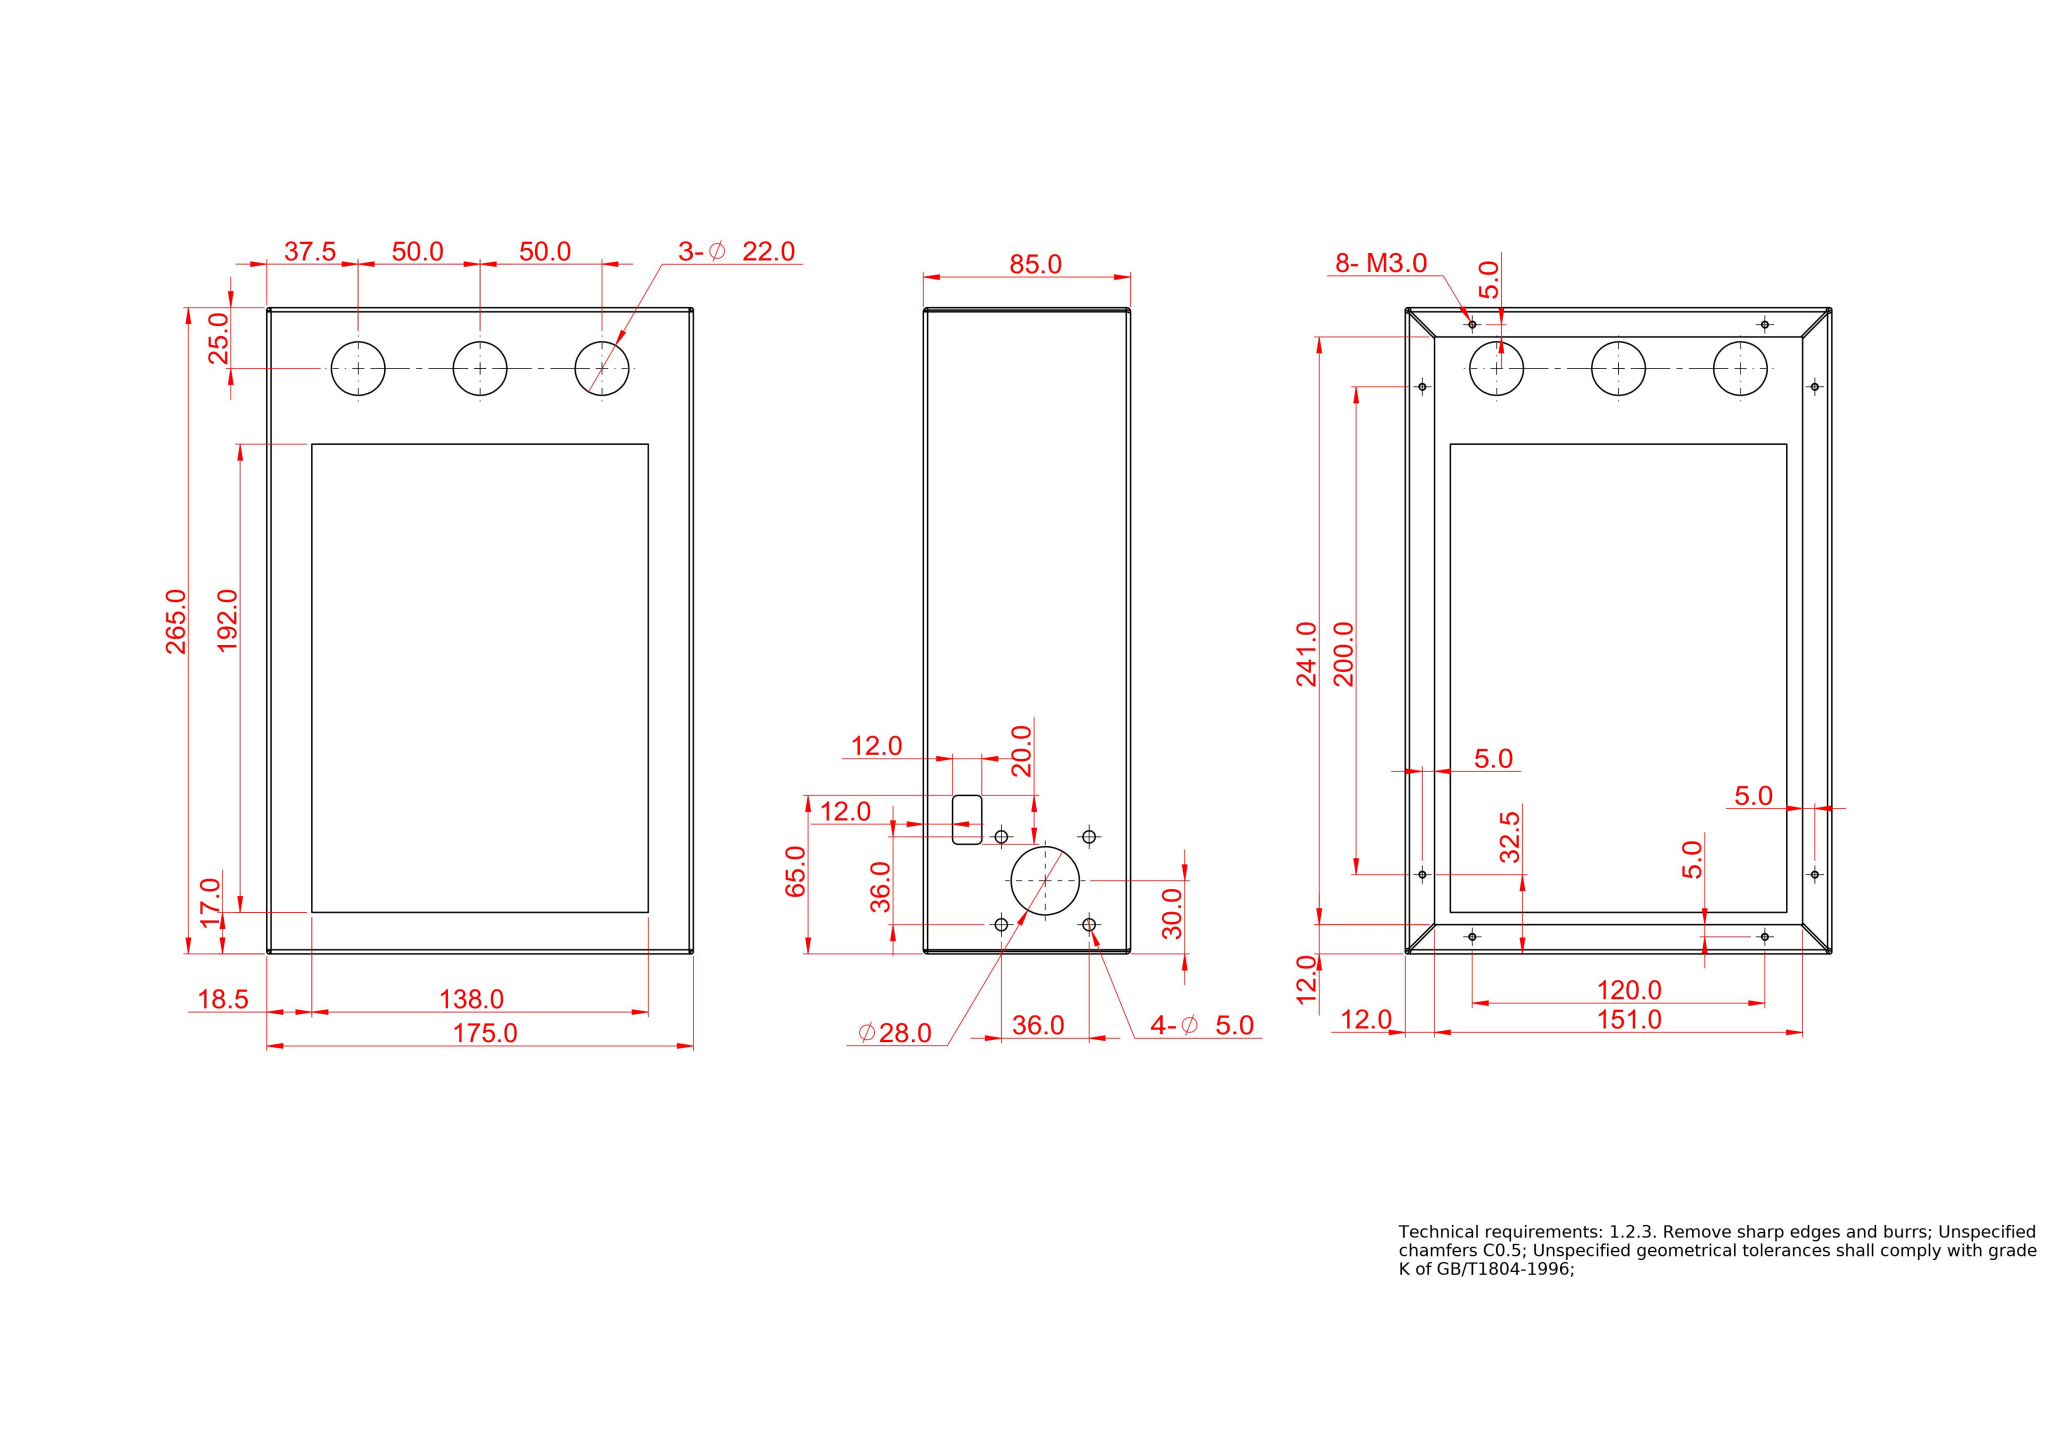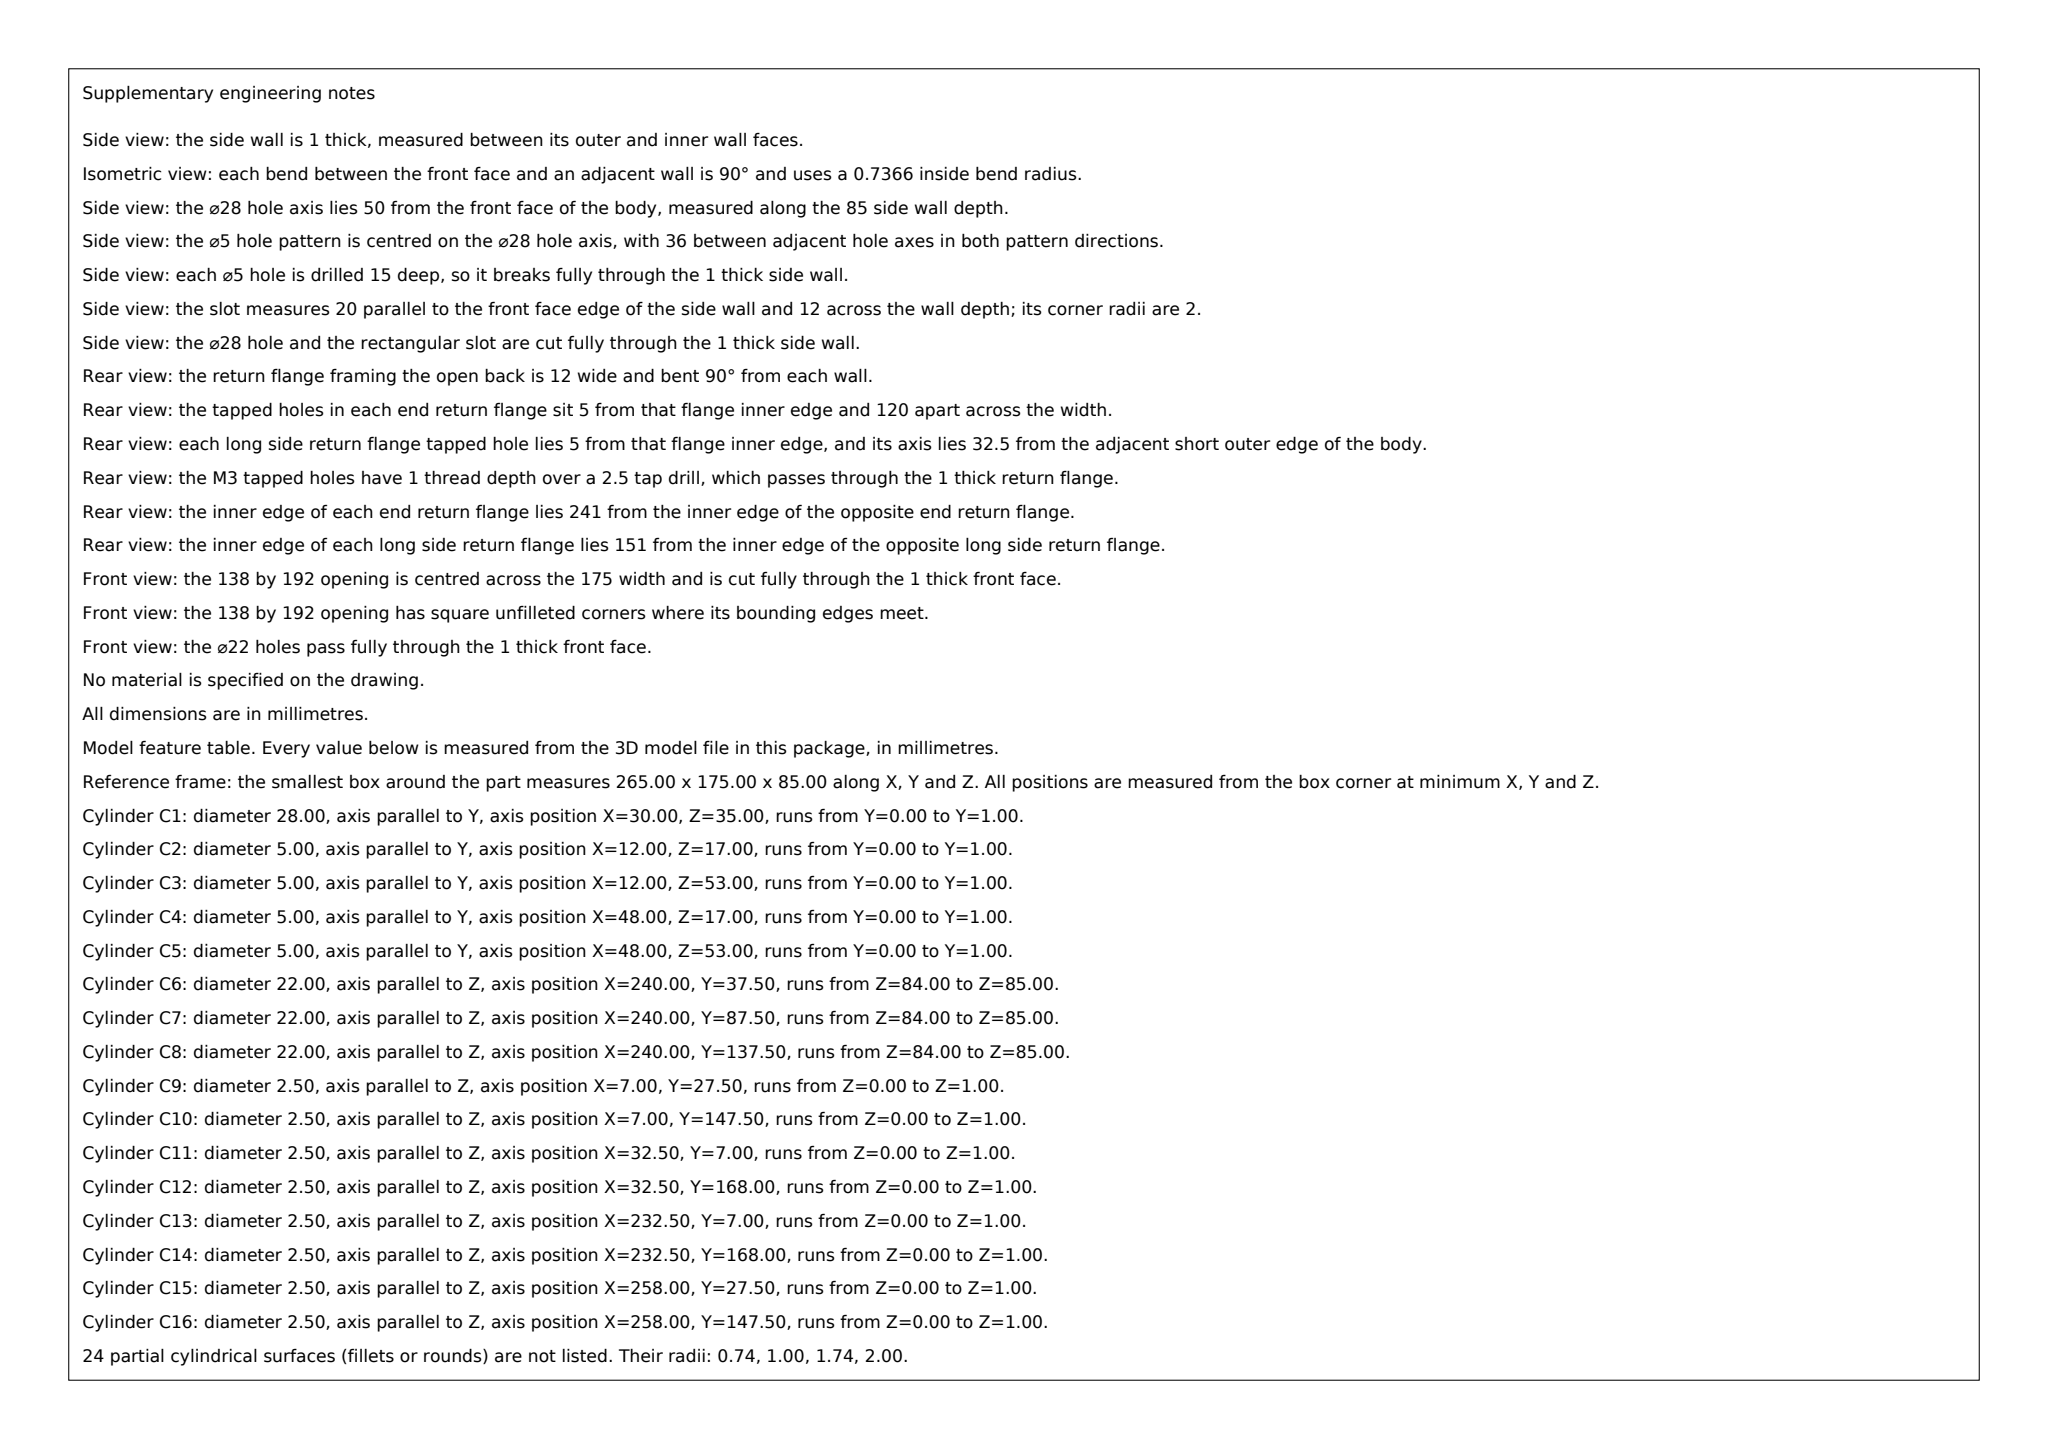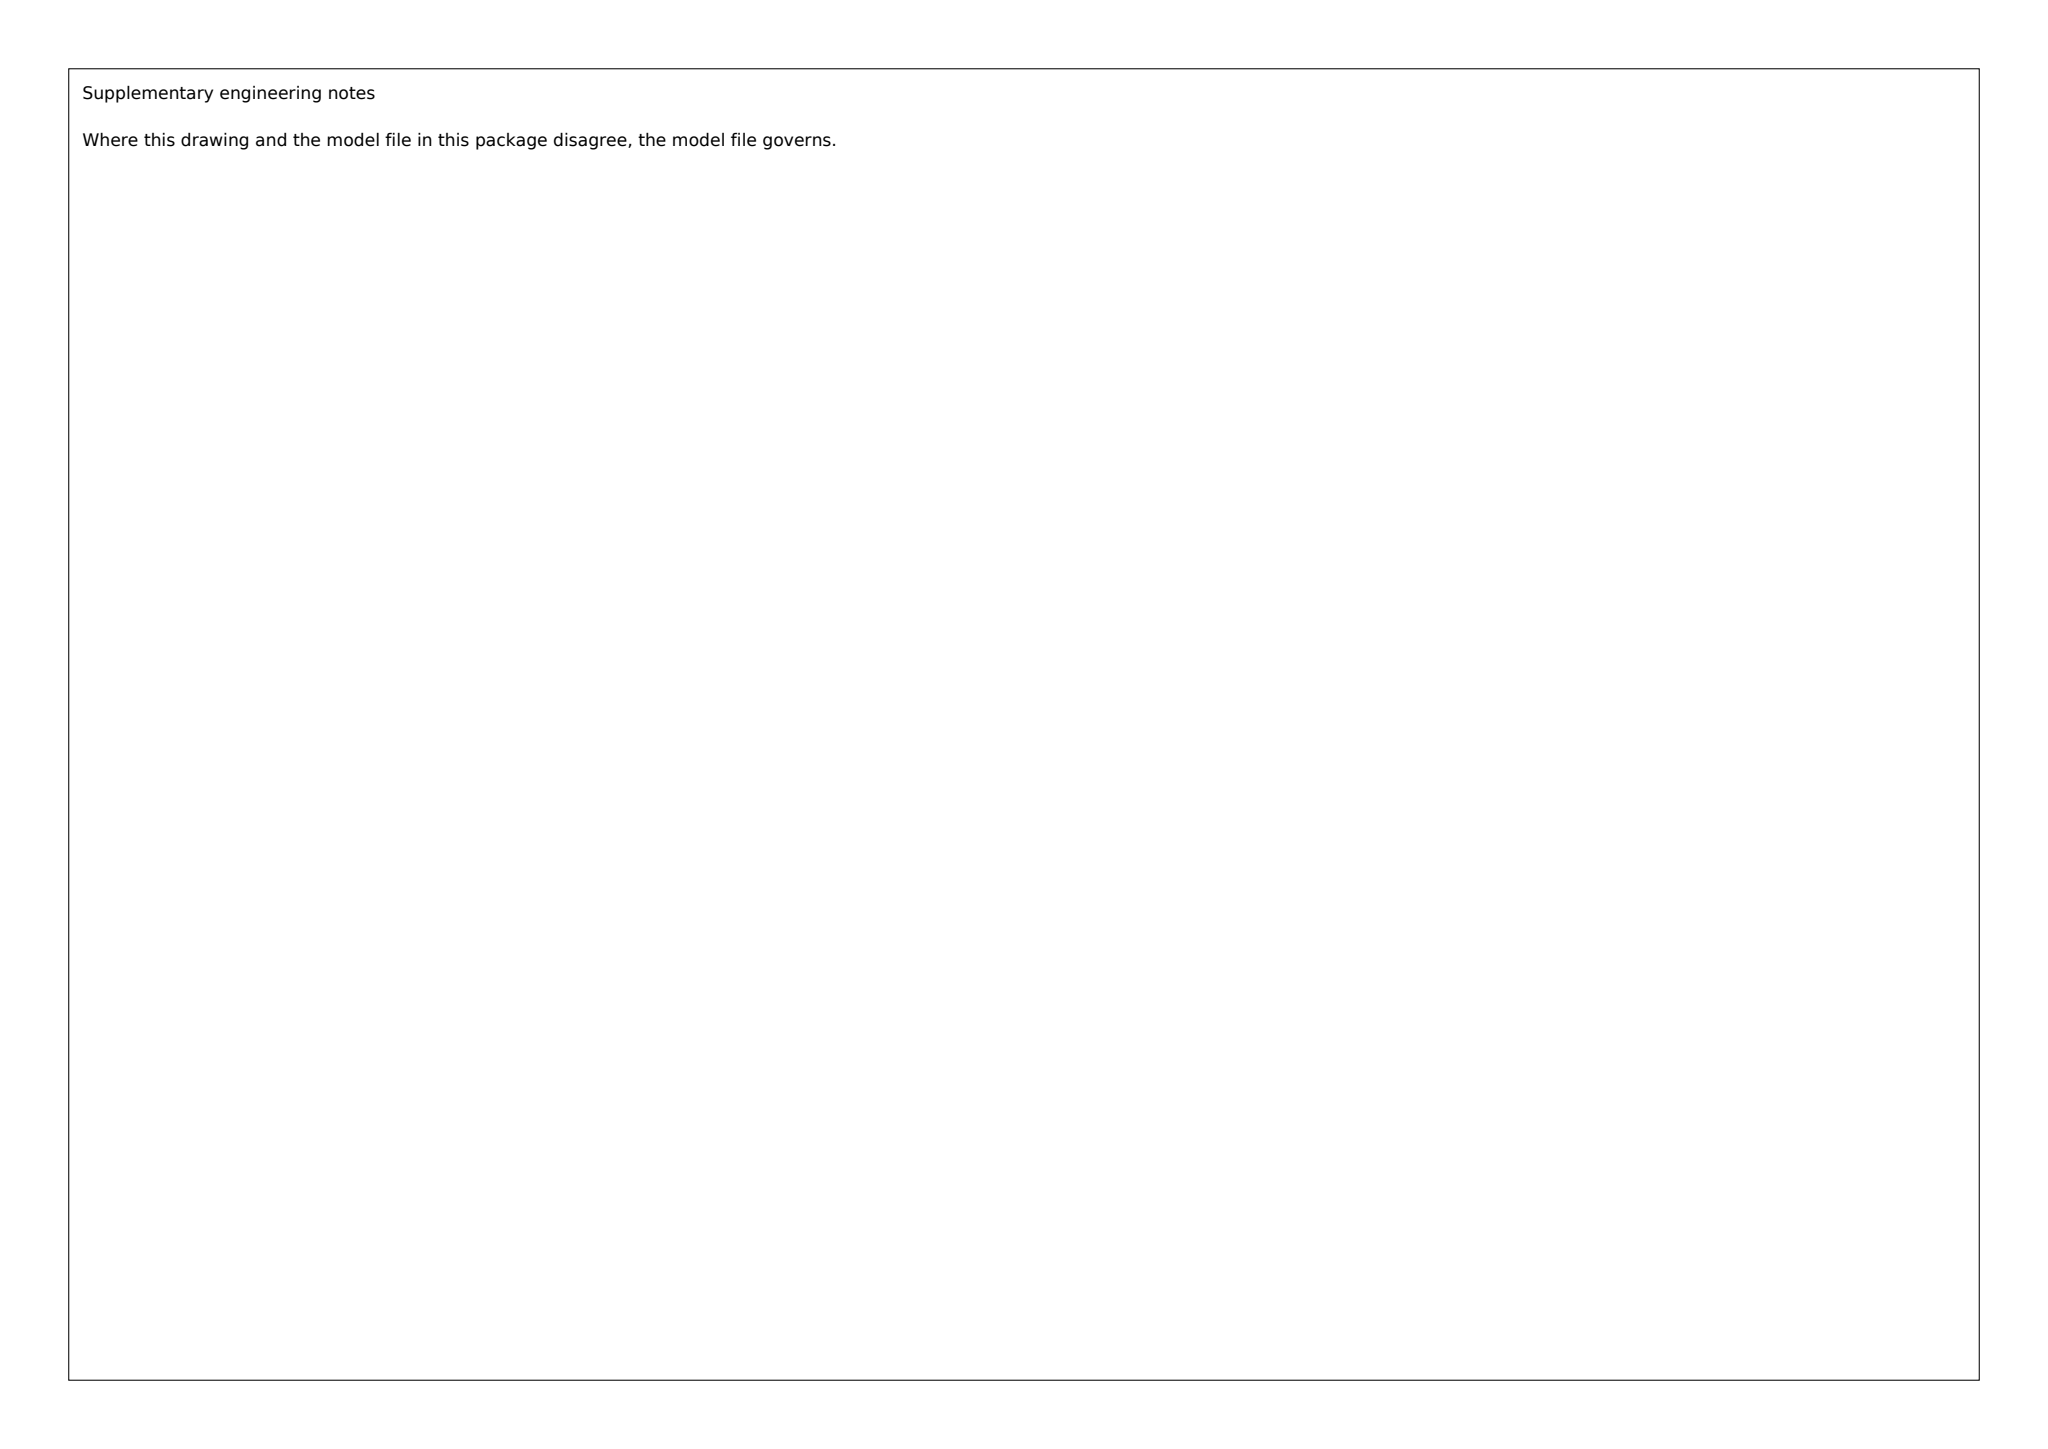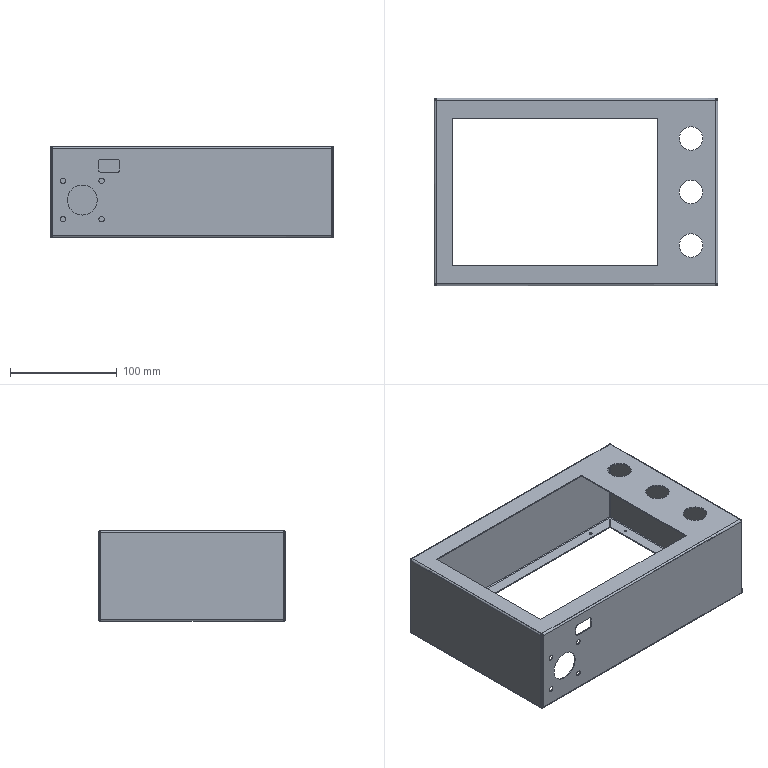Part | SolidWorks | mm | 1 solid | 158 faces | box 265 x 175 x 85 mm | volume 99459 mm3 | plane 62 | cylinder 56 | spline 40 | commonest cylinder face diameters 2.5 x16 5 x8 3.473 x8 1.473 x8 22 x6 2 x4 4 x4 28 x2
Drawing notes:
SHEET BENDS: INSIDE R0.74, OUTSIDE R1.74, MAT'L THK 1.0 | from the solid: Ø1.473 bend cyls at 1.74 offsets (R0.74 inner) & Ø3.473 (R1.74 outer); wall planes 0/1.0 apart
4X R1.0 ON VERT BOX CORNERS, FULL HT | from the solid: Ø2.0 z-axis cyls at (1,1),(1,174),(264,1),(264,174), L=81.53
8X M3.0 THRU 1.0 THK WALL | from the solid: 8X Ø2.5 z-axis holes, length 1.0 = wall thickness (planes z=0 to 1.0)